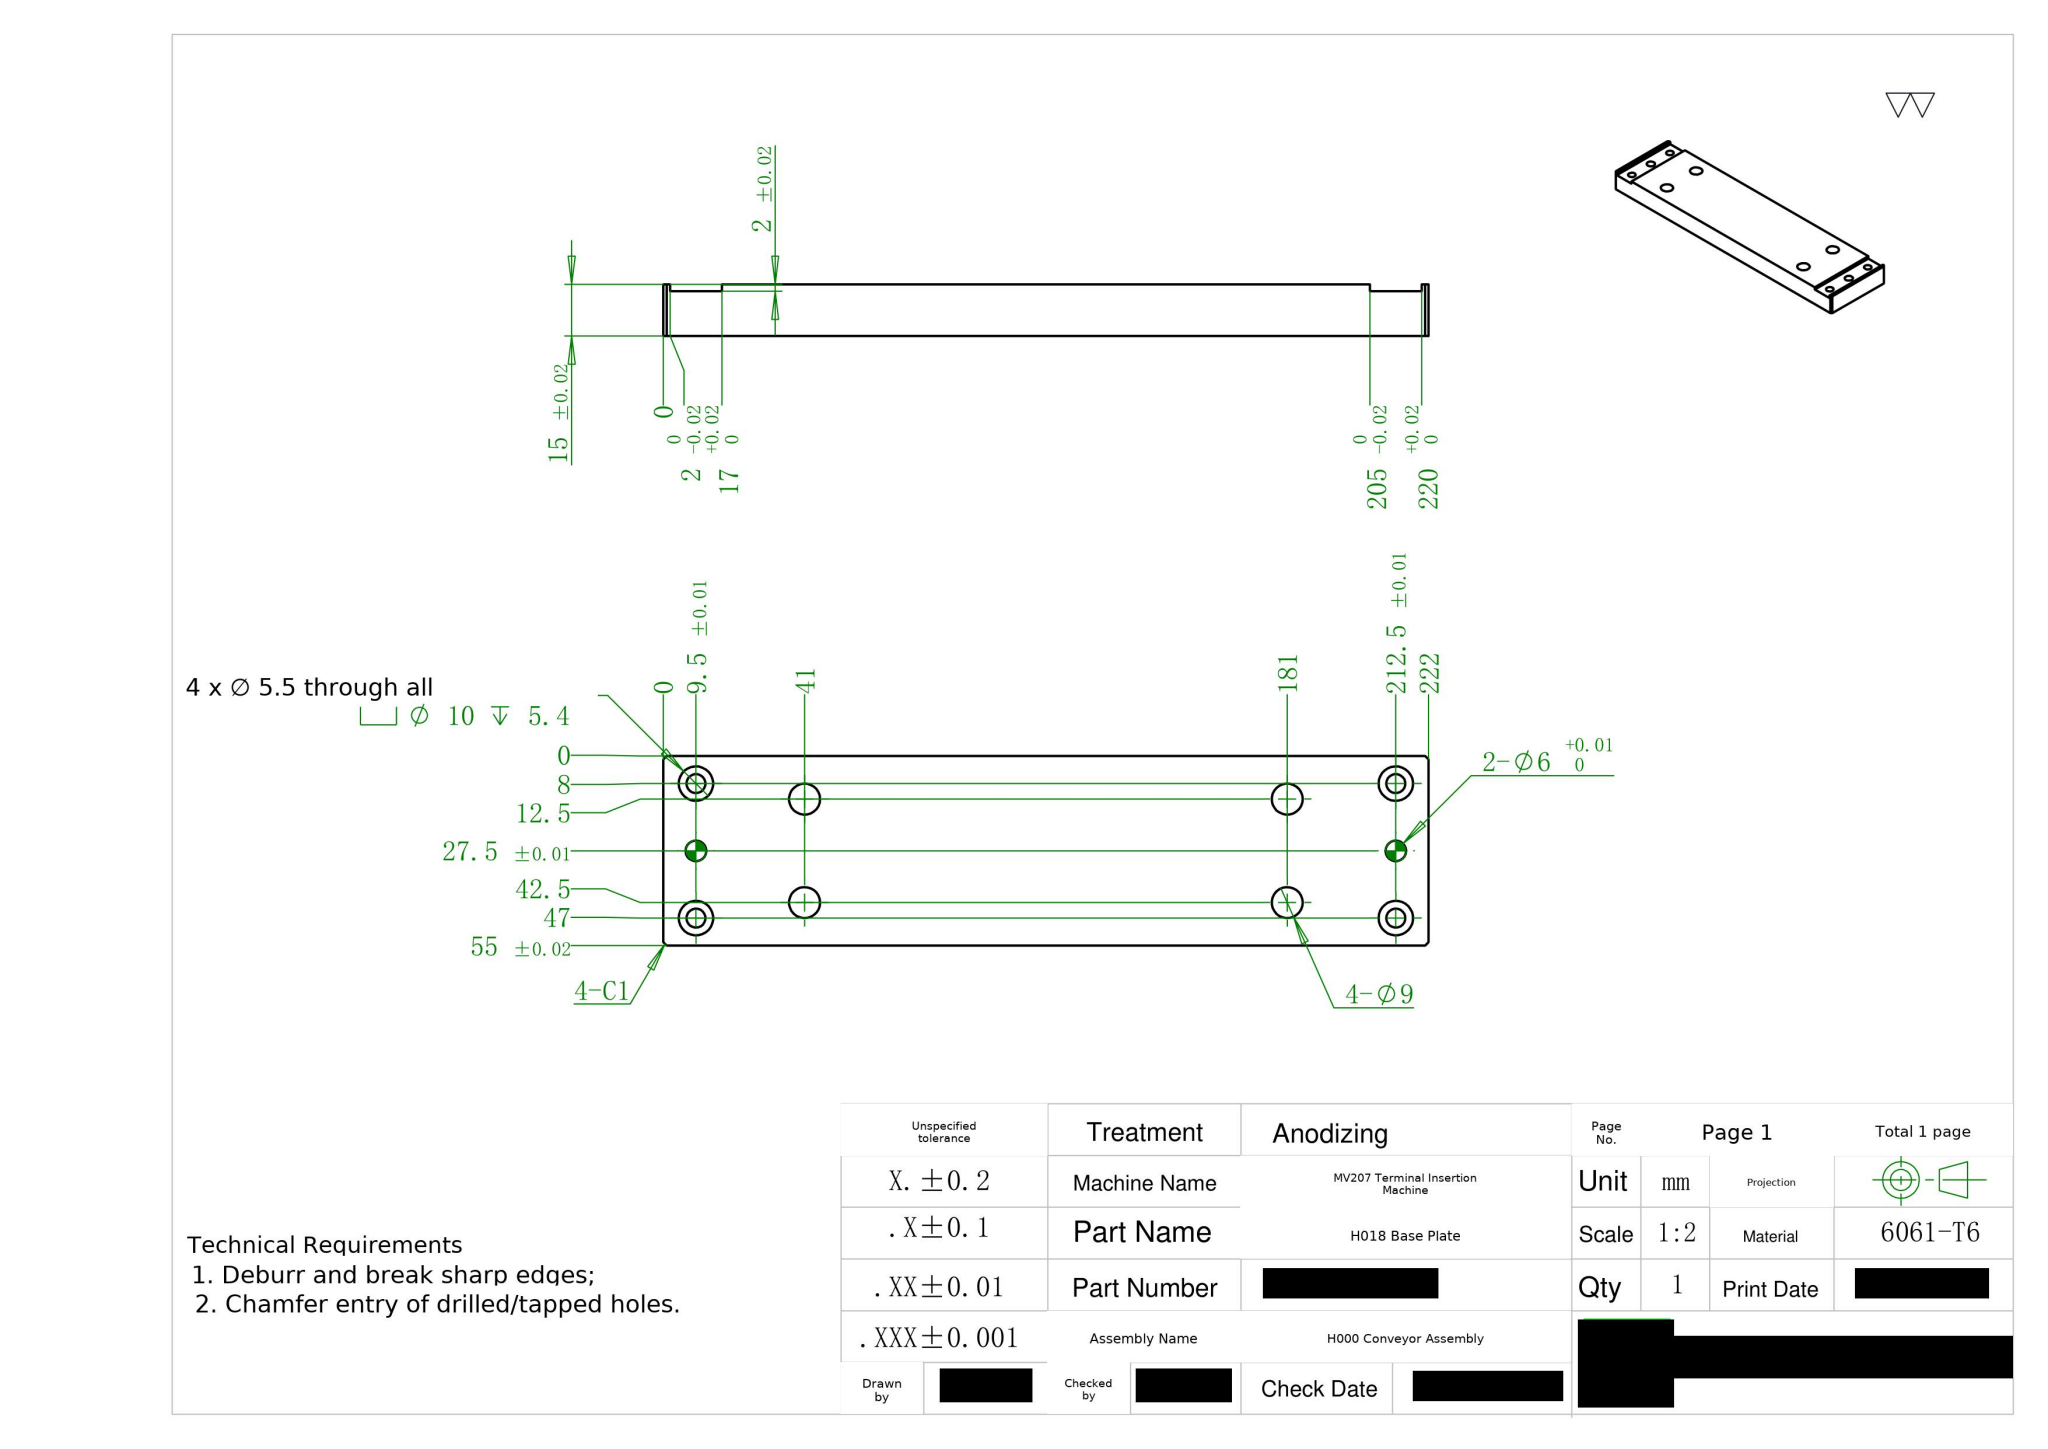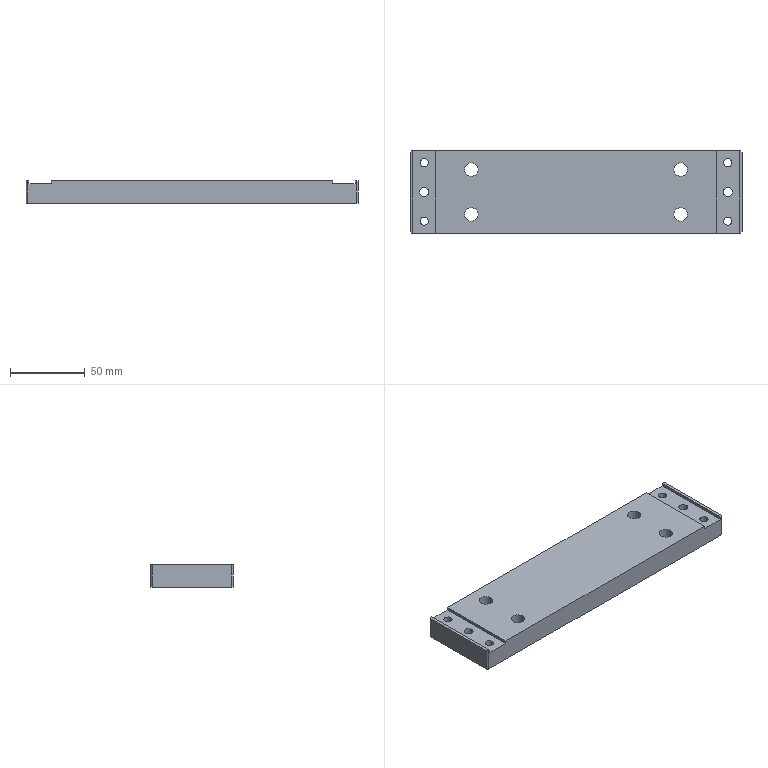Part | SolidWorks | mm | material 6061-T6 | 1 solid | 50 faces | box 222 x 55 x 15 mm | volume 172849 mm3 | cylinder 28 | plane 22 | commonest cylinder face diameters 10 x8 5.5 x8 9 x8 6 x4
build123d program:
from build123d import *

# Parameters (mm, degrees)
SKETCH1_W                                       = 222
SKETCH1_H                                       = 55
BOSS_EXTRUDE1_DEPTH                             = 15
CHAMFER1_SIZE                                   = 1
SKETCH4_W                                       = 15
SKETCH4_H                                       = 2
CUT_EXTRUDE1_DEPTH                              = 55
F_9_0_9_DIAMETER_HOLE1_D                        = 9
M5_HEX_SOCKET_HEAD_CAP_SCREW_CBORE1_D           = 5.5
M5_HEX_SOCKET_HEAD_CAP_SCREW_CBORE1_CBORE_D     = 10
M5_HEX_SOCKET_HEAD_CAP_SCREW_CBORE1_CBORE_DEPTH = 5.4
F_6_0_6_DIAMETER_HOLE1_D                        = 6


with BuildPart() as part:
    # Sketch1 → Boss-Extrude1 (new body)
    with BuildSketch(Plane.XY):
        Rectangle(SKETCH1_W, SKETCH1_H)
    extrude(amount=BOSS_EXTRUDE1_DEPTH)

    # Chamfer1
    chamfer1_edges = [part.edges().sort_by_distance(p)[0] for p in [
        (111, -27.5, 7.5),
        (-111, -27.5, 7.5),
        (-111, 27.5, 7.5),
        (111, 27.5, 7.5),
    ]]
    chamfer(chamfer1_edges, length=CHAMFER1_SIZE)

    # Sketch4 → Cut-Extrude1 (cut)
    with BuildSketch(Plane(origin=(0, -27.5, 0), x_dir=(1, 0, 0), z_dir=(0, 1, 0))):
        with Locations((101.5, -14)):
            Rectangle(SKETCH4_W, SKETCH4_H)
        with Locations((-101.5, -14)):
            Rectangle(SKETCH4_W, SKETCH4_H)
    extrude(amount=CUT_EXTRUDE1_DEPTH, mode=Mode.SUBTRACT)

    # 9.0 _9_ Diameter Hole1 (through all)
    with Locations(Plane.XY.offset(15)):
        with Locations((70, -15), (-70, -15), (-70, 15), (70, 15)):
            Hole(F_9_0_9_DIAMETER_HOLE1_D / 2)

    # M5 Hex Socket Head Cap Screw CBORE1 (through all)
    with Locations(Plane(origin=(0, 0, 0), x_dir=(-1, 0, 0), z_dir=(0, 0, -1))):
        with Locations((-101.5, 19.5), (-101.5, -19.5), (101.5, -19.5), (101.5, 19.5)):
            CounterBoreHole(M5_HEX_SOCKET_HEAD_CAP_SCREW_CBORE1_D / 2, M5_HEX_SOCKET_HEAD_CAP_SCREW_CBORE1_CBORE_D / 2, M5_HEX_SOCKET_HEAD_CAP_SCREW_CBORE1_CBORE_DEPTH)

    # 6.0 _6_ Diameter Hole1 (through all)
    with Locations(Plane(origin=(0, 0, 0), x_dir=(-1, 0, 0), z_dir=(0, 0, -1))):
        with Locations((101.5, 0), (-101.5, 0)):
            Hole(F_6_0_6_DIAMETER_HOLE1_D / 2)


solid = part.part